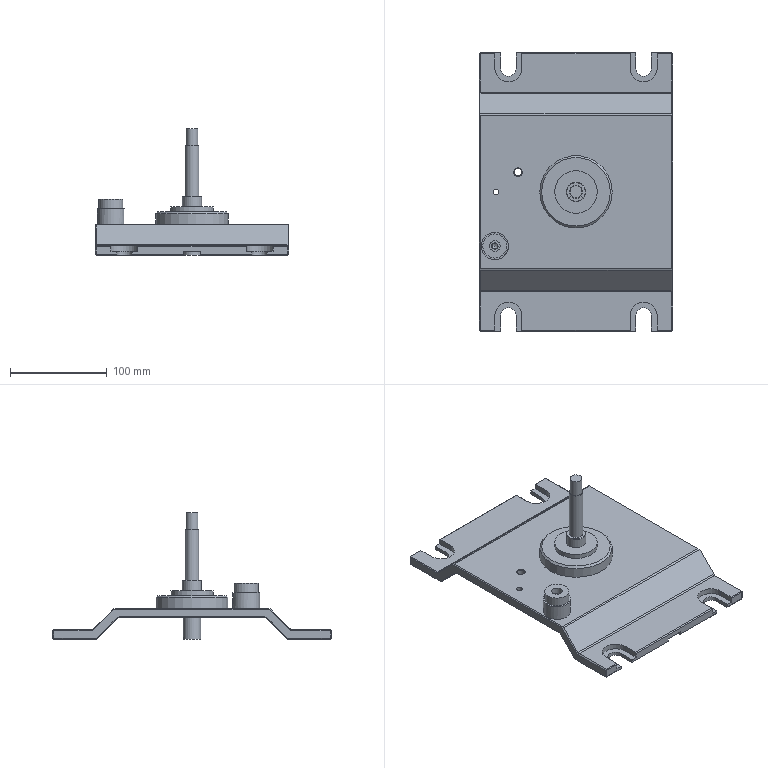Component | NX | Root-owned geometry | 3 solids | 150 faces | volume 677102 mm3 | plane 122 | cylinder 23 | cone 5 | commonest cylinder face diameters 28 x5 16 x4 20 x3 6 x2 75 x1 8 x1 14 x1 44 x1